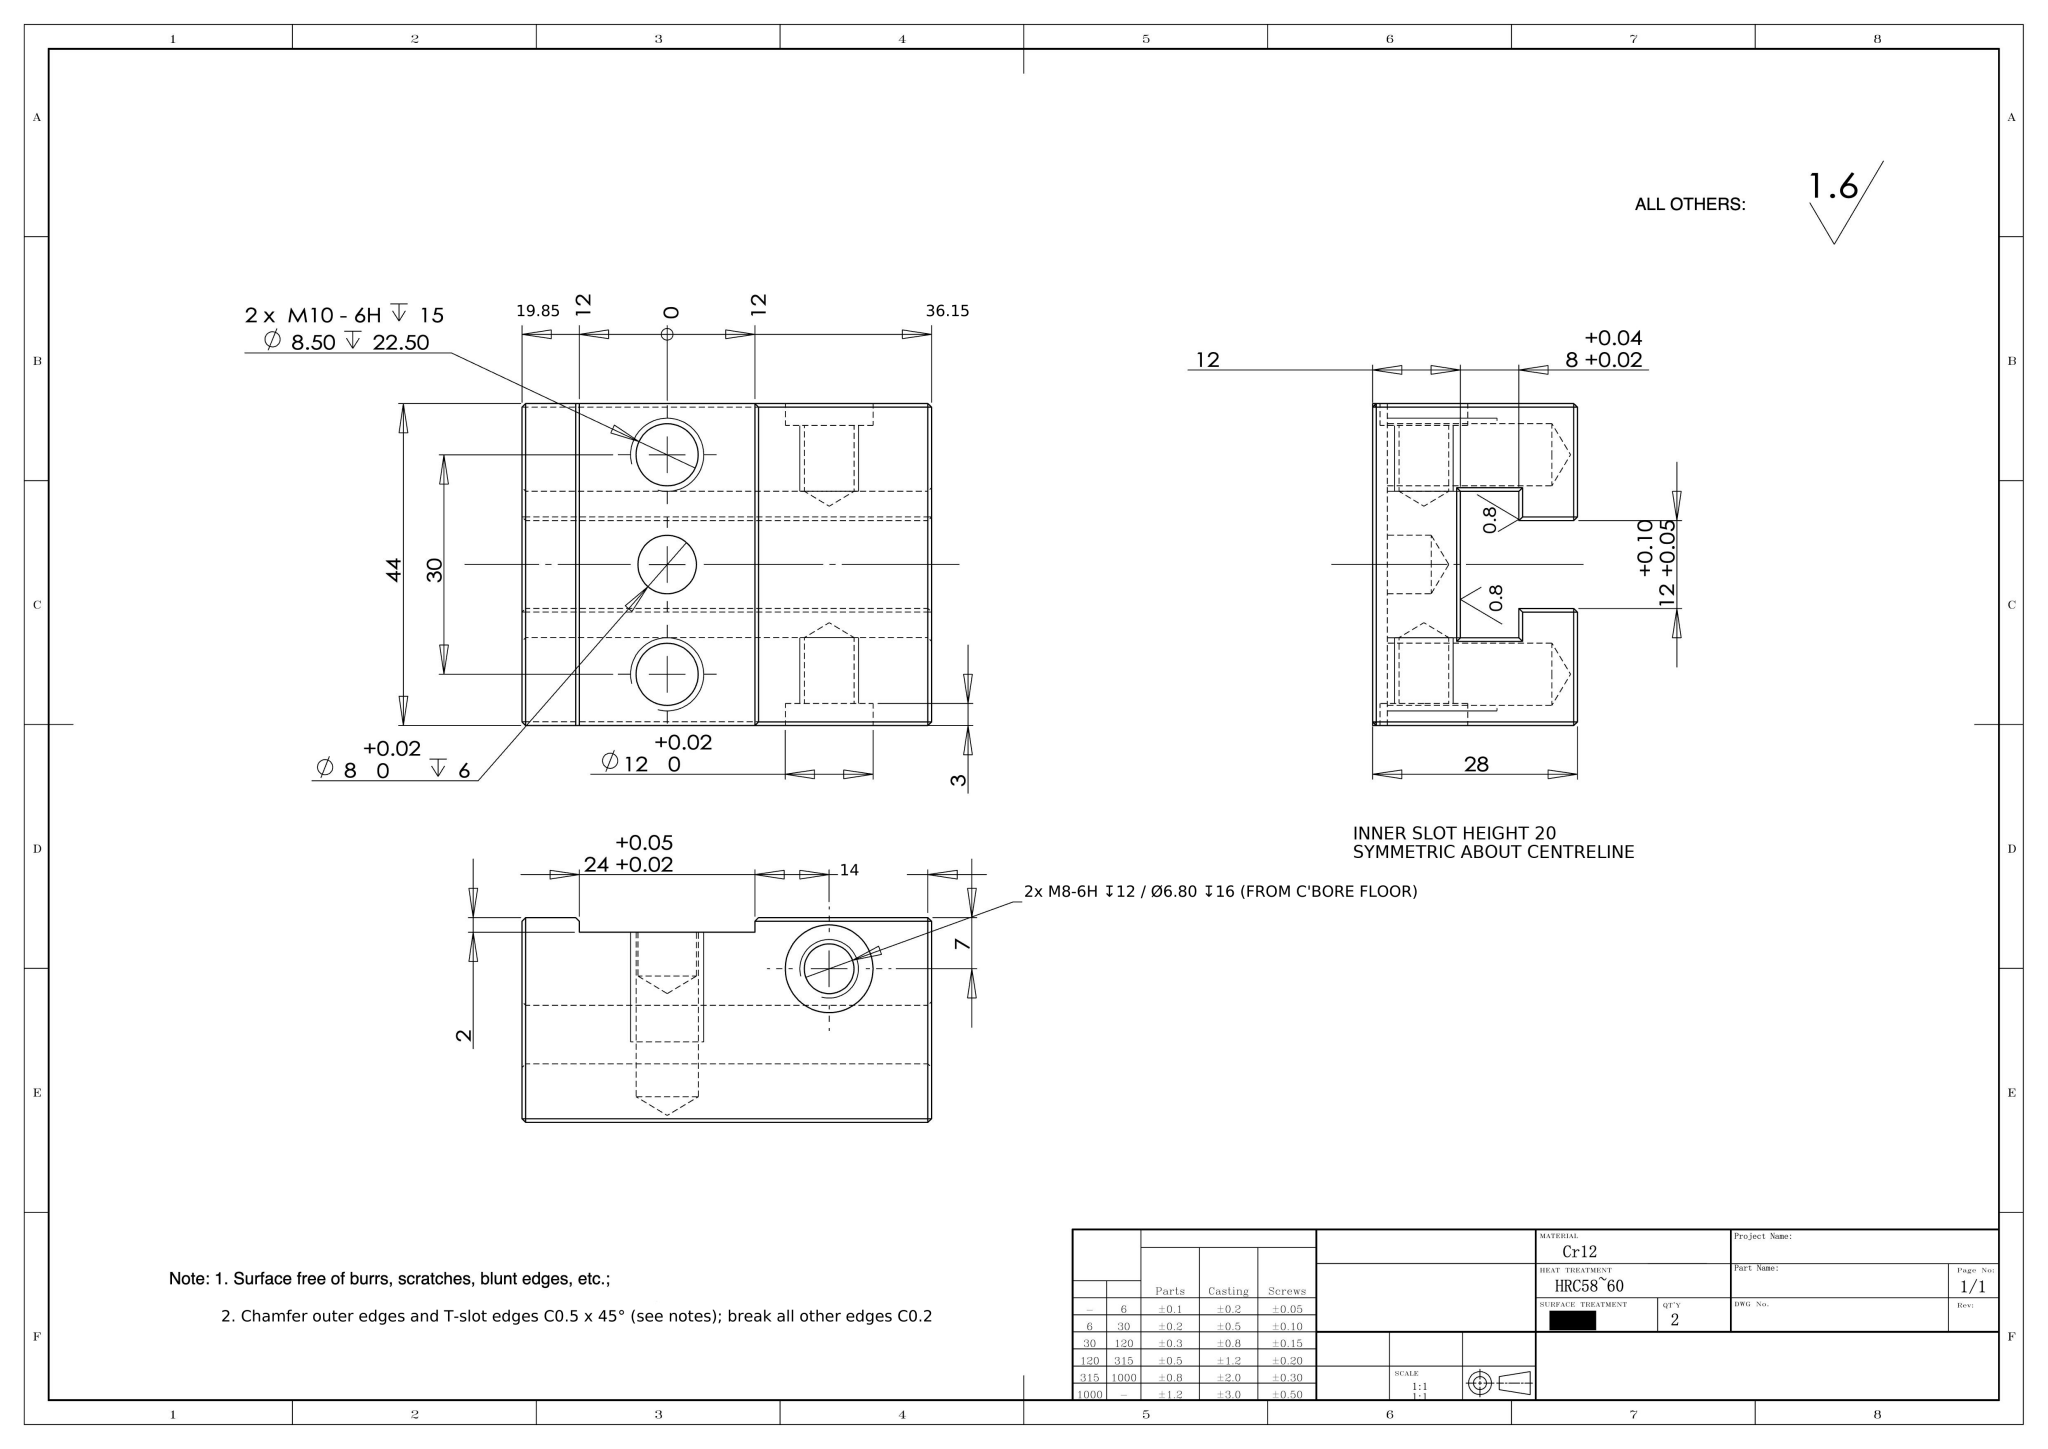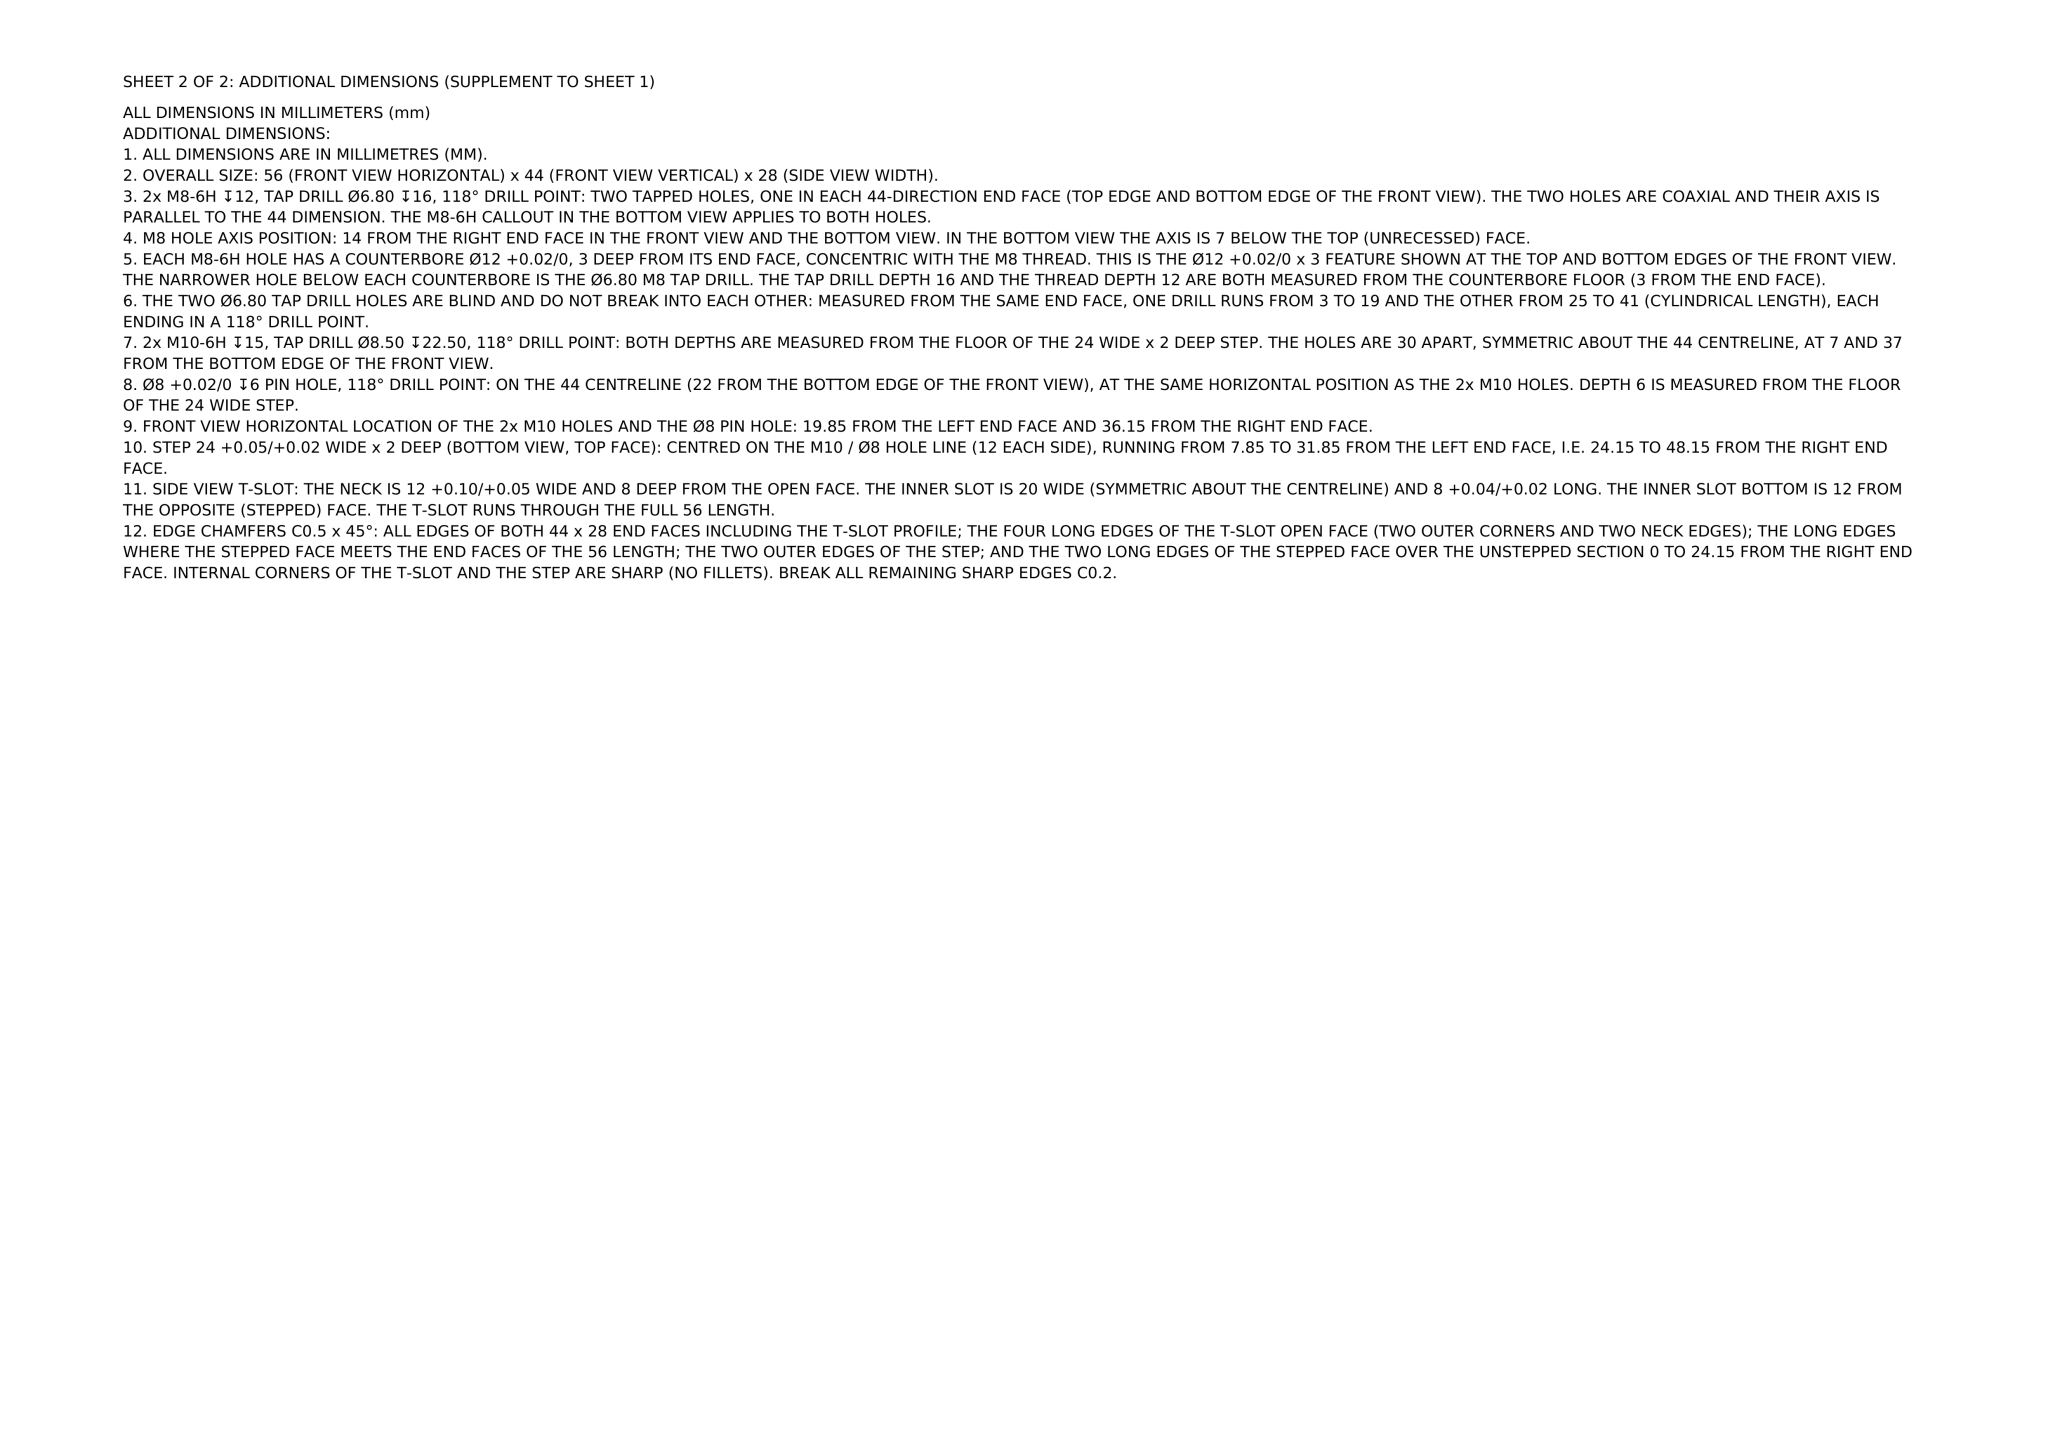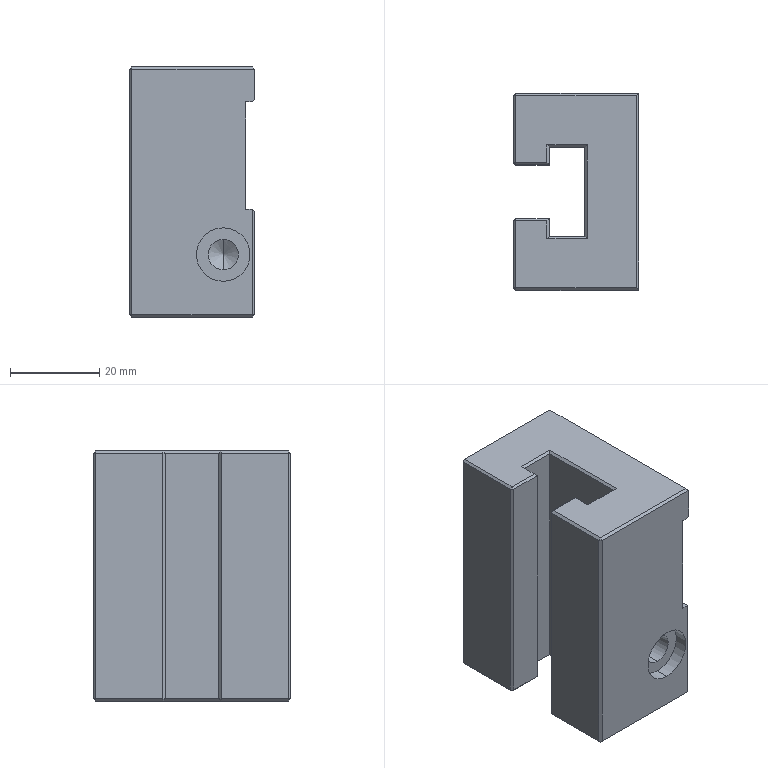Part | NX | mm | 1 solid | 86 faces | box 28 x 44 x 56 mm | volume 48078 mm3 | plane 62 | cylinder 14 | cone 10 | commonest cylinder face diameters 8.5 x4 6.8 x4 12 x4 8 x2